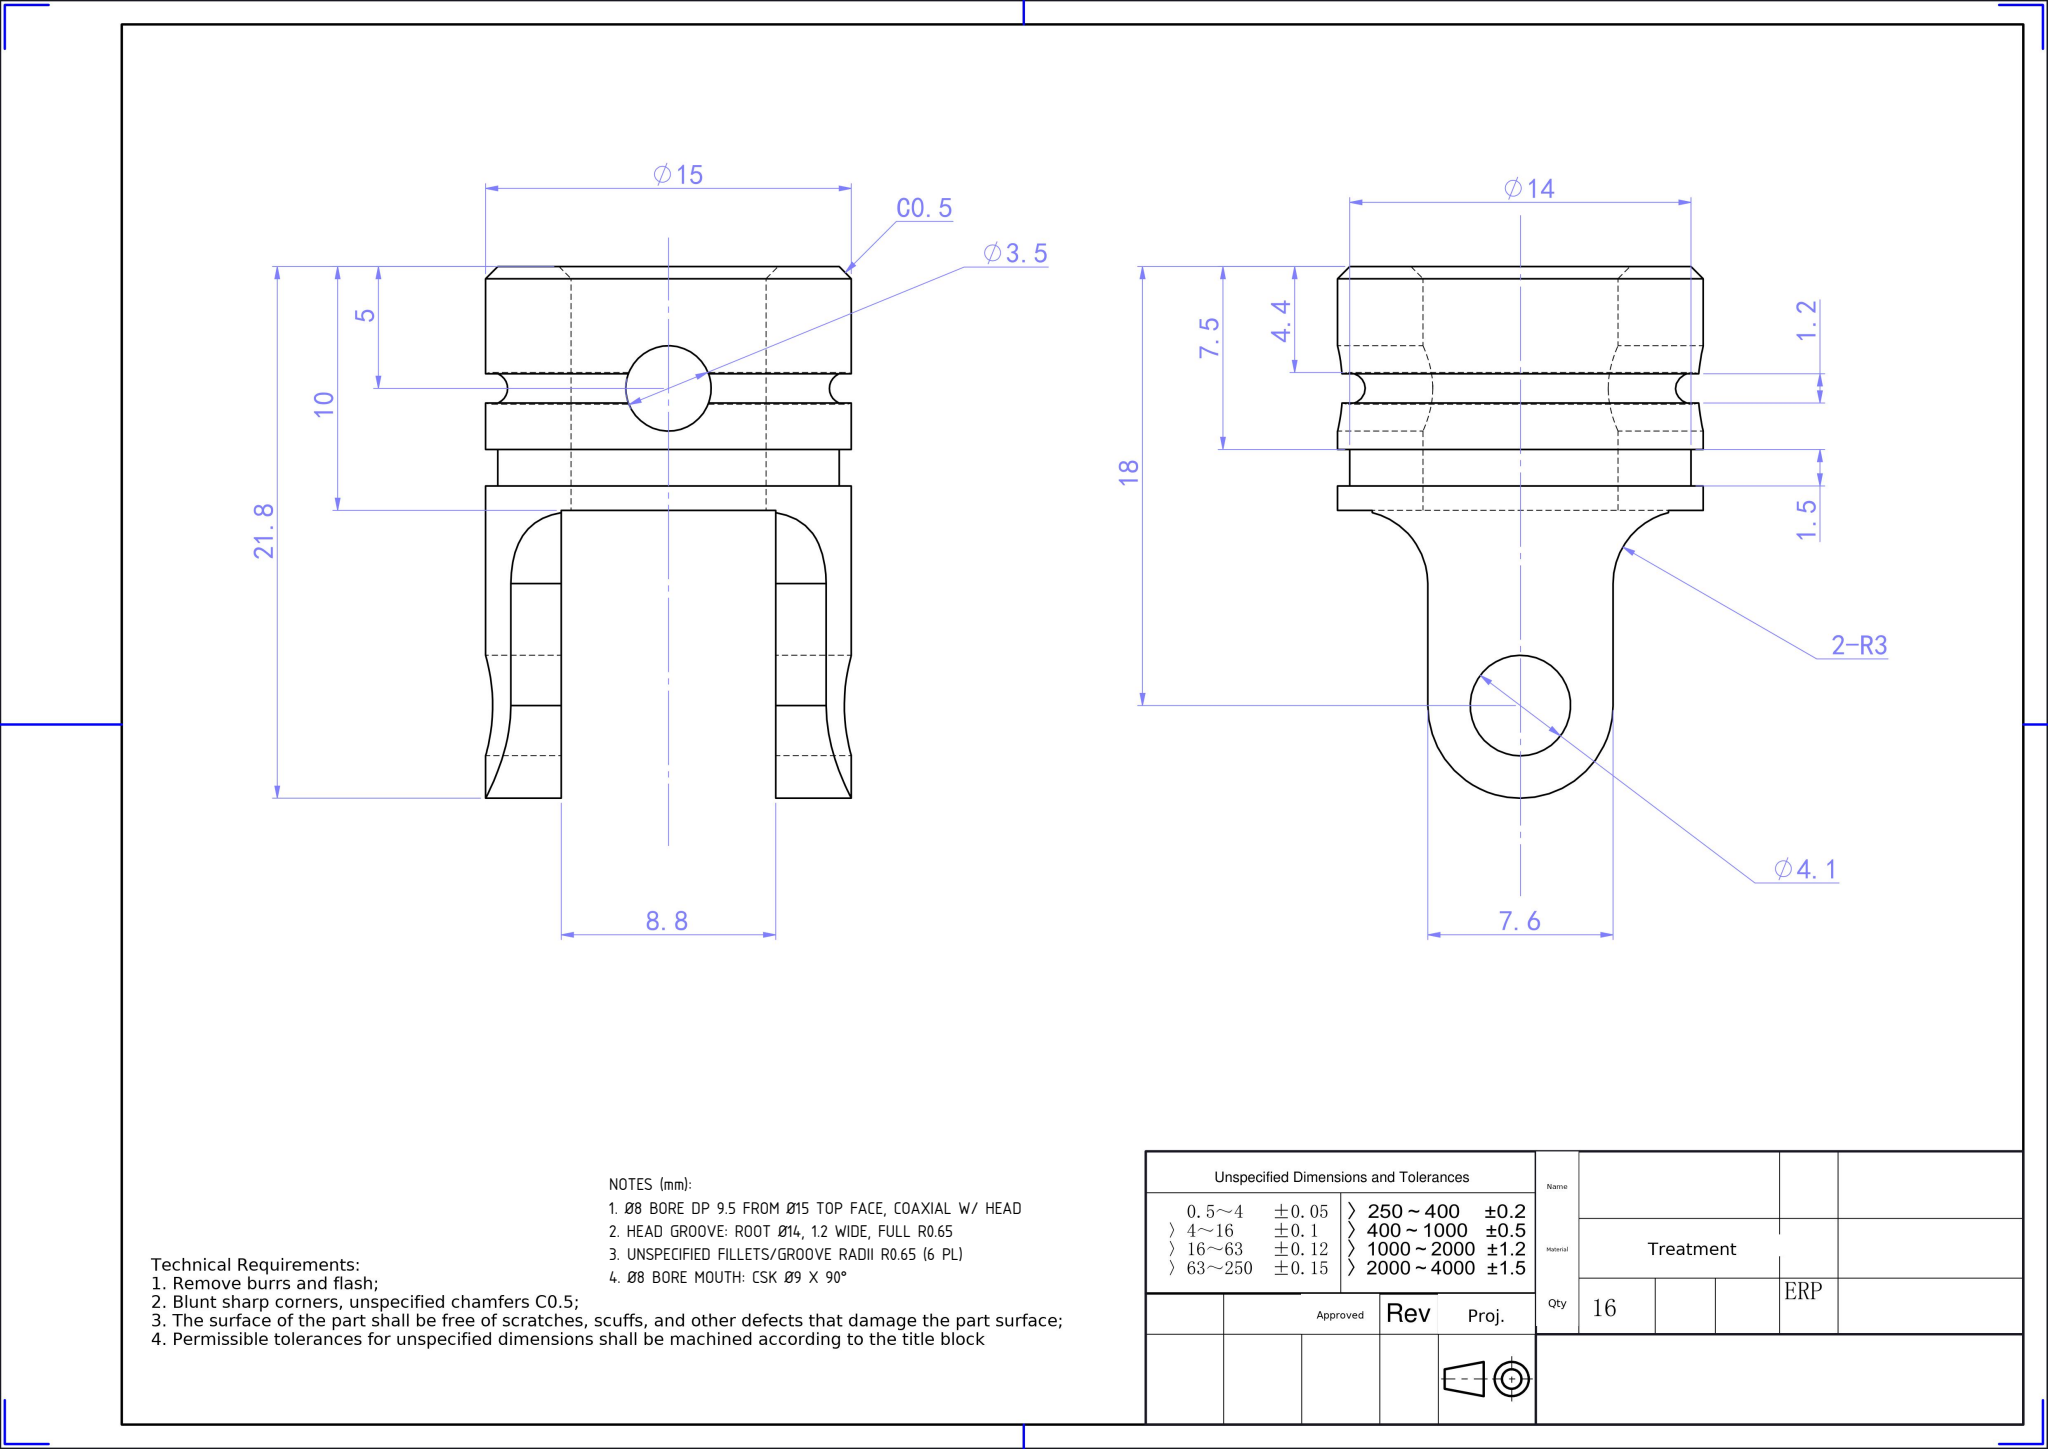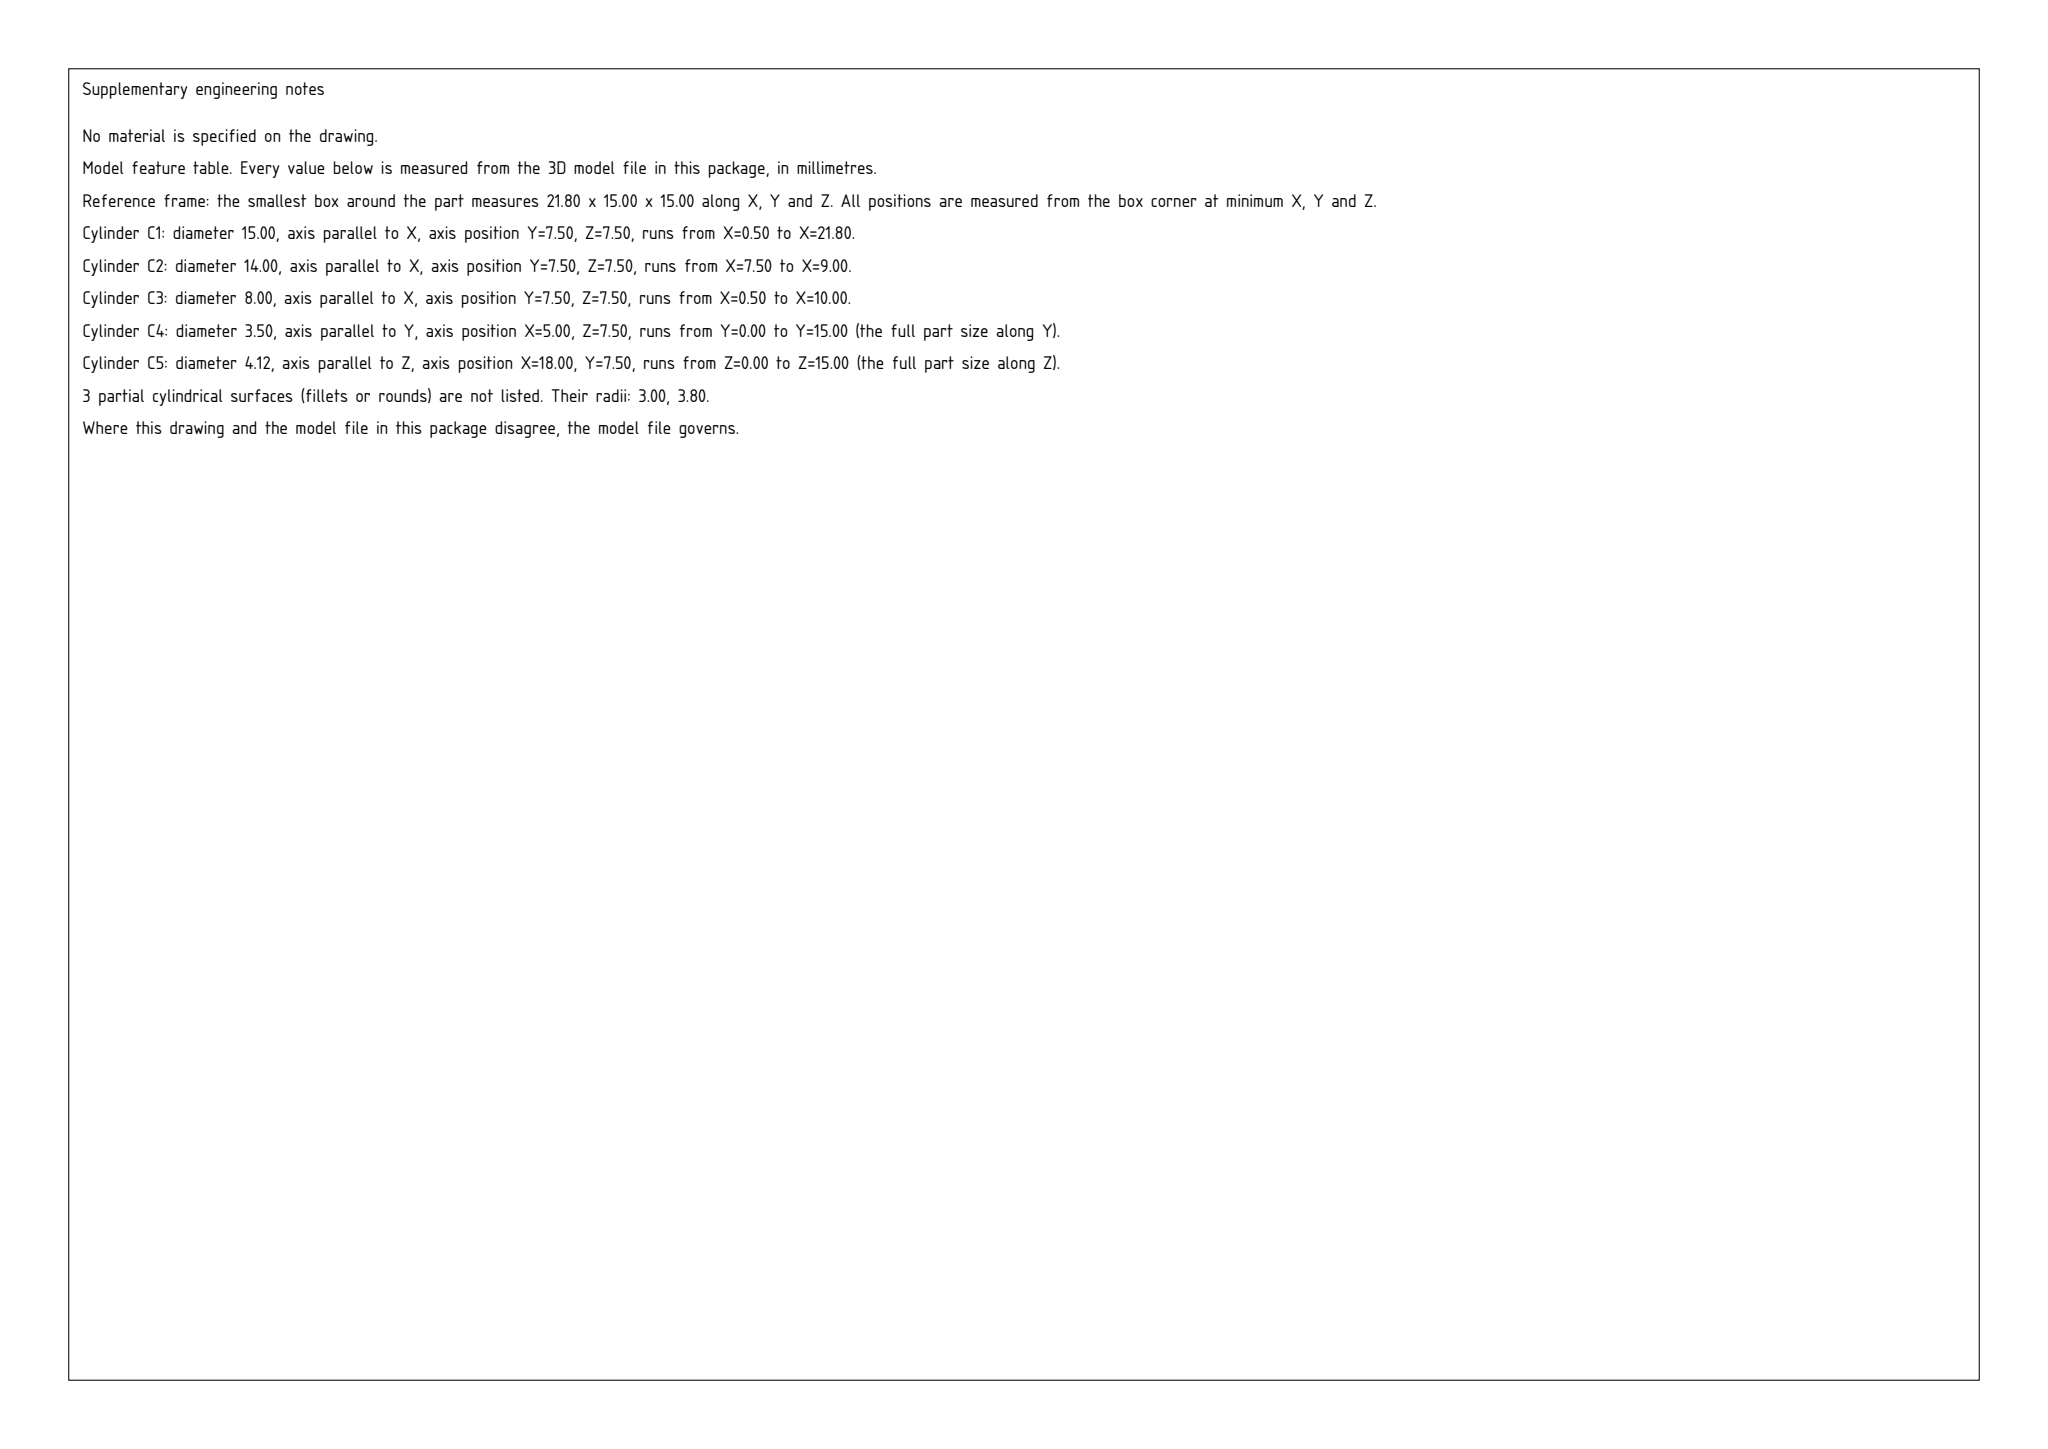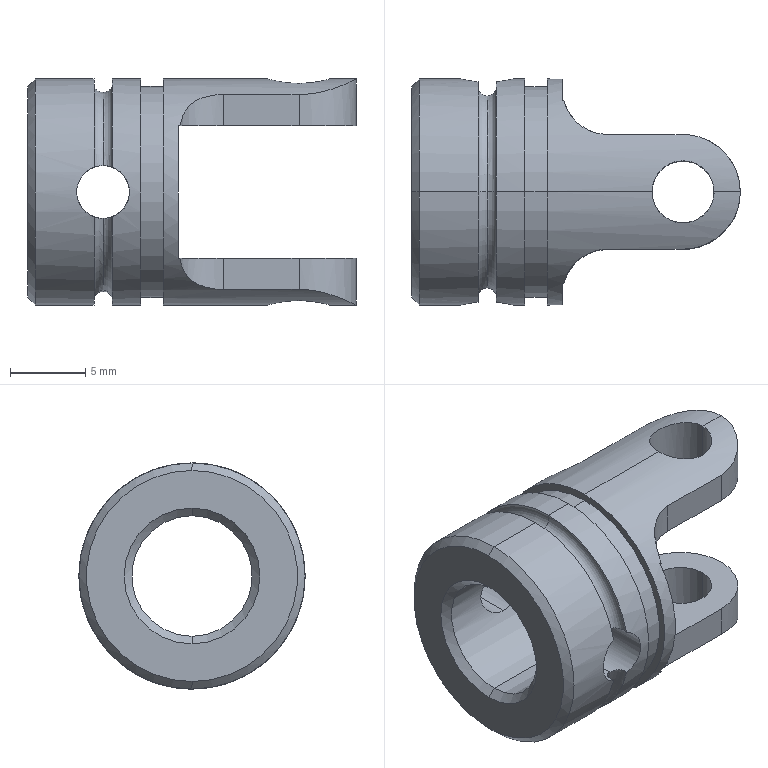Part | SolidWorks | mm | 1 solid | 46 faces | box 21.8 x 15 x 15 mm | volume 1513 mm3 | cylinder 26 | plane 10 | torus 6 | cone 4 | commonest cylinder face diameters 15 x6 3.5 x4 4.12 x4 7.6 x4 6 x4 14 x2 8 x2
Drawing notes:
Ø8 BORE DP 9.5 FROM Ø15 TOP FACE, COAXIAL W/ HEAD | from the solid: cylinder dia 8.0 axis x at (y 8.14, z 8.35), length 9.5, from x=0 face
HEAD GROOVE: ROOT Ø14, 1.2 WIDE, FULL R0.65 | from the solid: cylinder dia 14.0 axis x length 1.5 between Ø15 bands; fillet_radii 0.65
UNSPECIFIED FILLETS/GROOVE RADII R0.65 (6 PL) | from the solid: fillet_radii [[0.65, 6]]
Ø8 BORE MOUTH: CSK Ø9 X 90° | from the solid: cones [90.0 incl angle, ref dia 9.0, 2] at x=9.0 plane / bore entry
build123d program:
from build123d import *

# Parameters (mm, degrees)
CUT_EXTRUDE1_DEPTH      = 15
CUT_EXTRUDE1_DEPTH_BACK = 15
CUT_EXTRUDE2_DEPTH      = 15
CUT_EXTRUDE2_DEPTH_BACK = 15
SKETCH3_W               = 18
SKETCH3_H               = 8.8
SKETCH4_W               = 15
SKETCH4_H               = 2.06
SKETCH5_W               = 1.75
SKETCH5_H               = 15


with BuildPart() as part:
    # Sketch1 → Revolve1 (revolve)
    with BuildSketch(Plane.XY, mode=Mode.PRIVATE) as revolve1_sk:
        with BuildLine():
            Line((0, 7), (0, 4.5))
            Line((0, 4.5), (0.5, 4))
            Line((0.5, 4), (21.8, 4))
            Line((21.8, 4), (21.8, 7.5))
            Line((21.8, 7.5), (9, 7.5))
            Line((9, 7.5), (9, 7))
            Line((9, 7), (7.5, 7))
            Line((7.5, 7), (7.5, 7.5))
            Line((7.5, 7.5), (5.6, 7.5))
            ThreePointArc((5.6, 7.5), (5, 6.6), (4.4, 7.5))
            Line((4.4, 7.5), (0.5, 7.5))
            Line((0.5, 7.5), (0, 7))
        make_face()
    revolve(revolve1_sk.sketch.rotate(Axis((21.8, 0, 0), (-1, 0, 0)), 270), axis=Axis((21.8, 0, 0), (-1, 0, 0)))

    # Sketch2 → Cut-Extrude1 (cut, two sides: drawn at the far end of the back side and taken through both)
    with BuildSketch(Plane.XY.offset(-CUT_EXTRUDE1_DEPTH_BACK)):
        with BuildLine():
            Line((10, 8.5), (10, 6.8))
            ThreePointArc((10, 6.8), (10.879, 4.679), (13, 3.8))
            Line((13, 3.8), (18, 3.8))
            ThreePointArc((18, 3.8), (21.8, 0), (18, -3.8))
            Line((18, -3.8), (13, -3.8))
            ThreePointArc((13, -3.8), (10.879, -4.679), (10, -6.8))
            Line((10, -6.8), (10, -8.5))
            Line((10, -8.5), (28, -8.5))
            Line((28, -8.5), (28, 8.5))
            Line((28, 8.5), (10, 8.5))
        make_face()
    extrude(amount=CUT_EXTRUDE1_DEPTH + CUT_EXTRUDE1_DEPTH_BACK, mode=Mode.SUBTRACT)

    # Sketch3 → Cut-Extrude2 (cut, two sides: drawn at the far end of the back side and taken through both)
    with BuildSketch(Plane(origin=(0, 0, 0), x_dir=(1, 0, 0), z_dir=(0, 1, 0)).offset(-CUT_EXTRUDE2_DEPTH_BACK)):
        with Locations((19, 0)):
            Rectangle(SKETCH3_W, SKETCH3_H)
    extrude(amount=CUT_EXTRUDE2_DEPTH + CUT_EXTRUDE2_DEPTH_BACK, mode=Mode.SUBTRACT)

    # Sketch4 → Cut-Revolve1 (revolve, cut)
    with BuildSketch(Plane(origin=(18, 0, 0), x_dir=(0, 0, -1), z_dir=(1, 0, 0)), mode=Mode.PRIVATE) as cut_revolve1_sk:
        with Locations((0, 1.03)):
            Rectangle(SKETCH4_W, SKETCH4_H)
    revolve(cut_revolve1_sk.sketch.rotate(Axis((18, 0, -7.5), (0, 0, 1)), 270), axis=Axis((18, 0, -7.5), (0, 0, 1)), mode=Mode.SUBTRACT)

    # Sketch5 → Cut-Revolve2 (revolve, cut)
    with BuildSketch(Plane(origin=(5, 0, 0), x_dir=(0, 0, -1), z_dir=(1, 0, 0)), mode=Mode.PRIVATE) as cut_revolve2_sk:
        with Locations((0.875, 0)):
            Rectangle(SKETCH5_W, SKETCH5_H)
    revolve(cut_revolve2_sk.sketch.rotate(Axis((5, -7.5, 0), (0, 1, 0)), 180), axis=Axis((5, -7.5, 0), (0, 1, 0)), mode=Mode.SUBTRACT)


solid = part.part